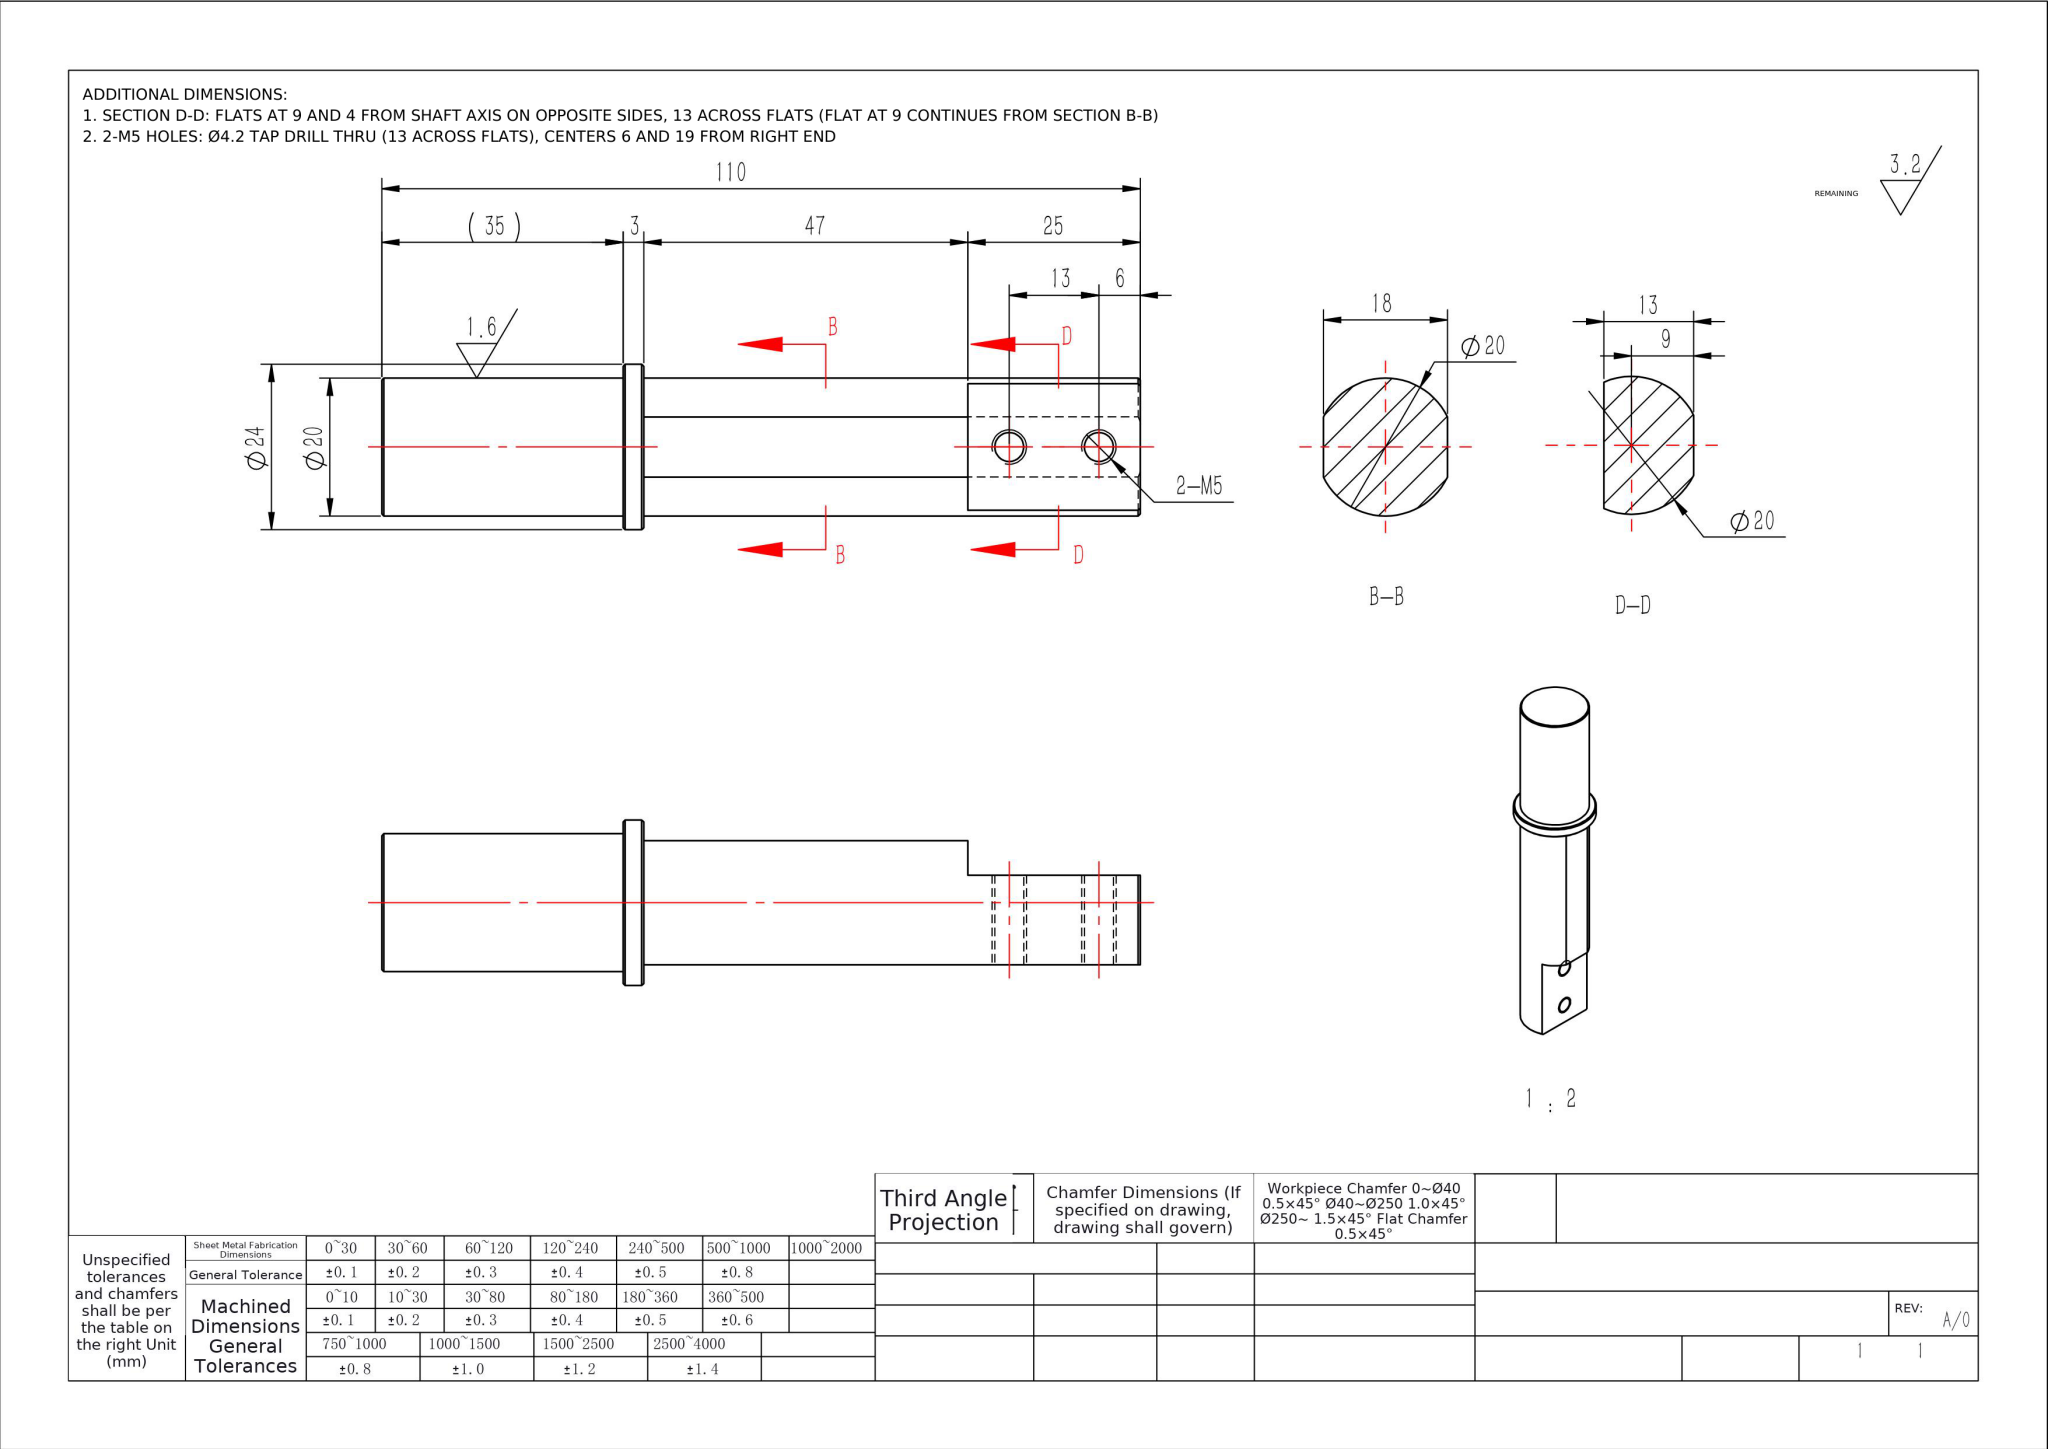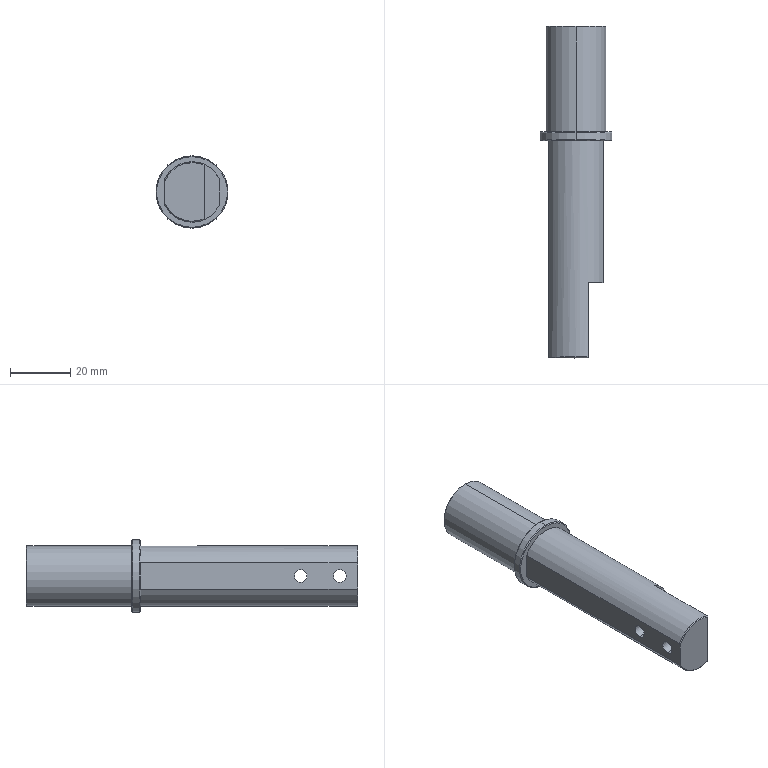Part | NX | mm | 1 solid | 28 faces | box 24 x 110 x 24 mm | volume 31921 mm3 | cylinder 11 | cone 9 | plane 8 | commonest cylinder face diameters 20 x5 4.2 x4 24 x2